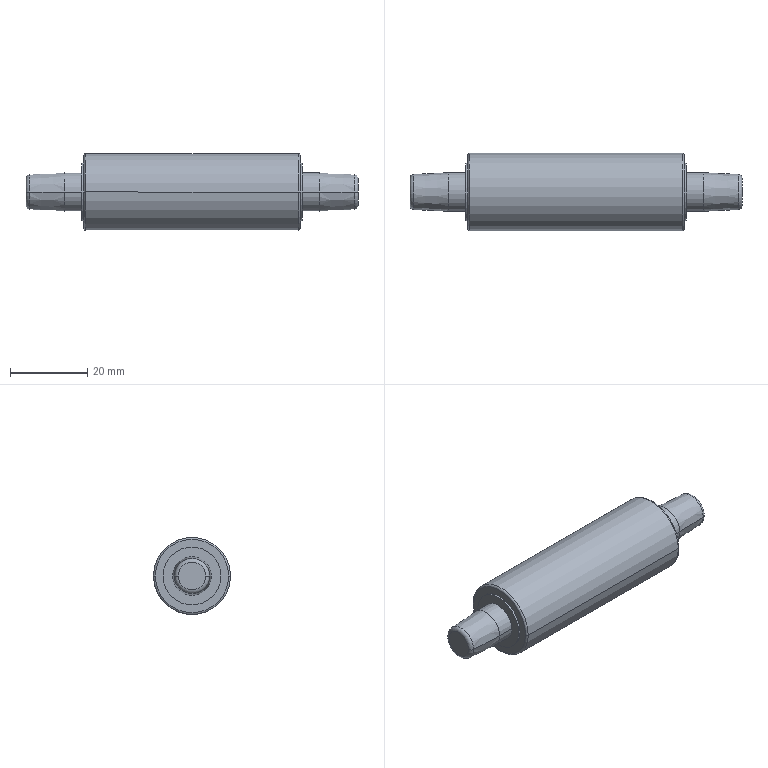Component | SolidWorks | RMS_20X400_03-1_RMS20X50_Piston-1 | 1 solid | 28 faces | box 86 x 20 x 20 mm | volume 19878 mm3 | cylinder 10 | torus 8 | plane 6 | cone 4 | commonest cylinder face diameters 10 x4 15 x4 20 x2
build123d program:
from build123d import *


with BuildPart() as part:
    # Sketch1 → Revolve1 (revolve)
    with BuildSketch(Plane.XY, mode=Mode.PRIVATE) as revolve1_sk:
        with BuildLine():
            Line((-15, 0), (-15, 3.549))
            ThreePointArc((-15, 3.549), (-14.725, 4.238), (-14.05, 4.548))
            Line((-14.05, 4.548), (-5, 5))
            Line((-5, 5), (-0.5, 5))
            Line((-0.5, 5), (-0.5, 7.5))
            Line((-0.5, 7.5), (0, 7.5))
            Line((0, 7.5), (0, 9.5))
            ThreePointArc((0, 9.5), (0.1464, 9.854), (0.5, 10))
            Line((0.5, 10), (55.5, 10))
            ThreePointArc((55.5, 10), (55.854, 9.854), (56, 9.5))
            Line((56, 9.5), (56, 7.5))
            Line((56, 7.5), (56.5, 7.5))
            Line((56.5, 7.5), (56.5, 5))
            Line((56.5, 5), (61, 5))
            Line((61, 5), (70.05, 4.548))
            ThreePointArc((70.05, 4.548), (70.725, 4.238), (71, 3.549))
            Line((71, 3.549), (71, 0))
            Line((71, 0), (-15, 0))
        make_face()
    revolve(revolve1_sk.sketch.rotate(Axis((71, 0, 0), (-1, 0, 0)), 270), axis=Axis((71, 0, 0), (-1, 0, 0)))


solid = part.part

# Placed as in the assembly
solid = solid.moved(Location((-0.1195, 21, 41.5), (0, 0, 0)))
STEP:
#1=CARTESIAN_POINT('',(2.791,0.9665,1.634));
#2=VERTEX_POINT('',#1);
#3=CARTESIAN_POINT('',(2.791,0.6871,1.634));
#4=VERTEX_POINT('',#3);
#5=CARTESIAN_POINT('',(2.791,0.8268,1.634));
#6=DIRECTION('',(-1.,0.,0.));
#7=DIRECTION('',(0.,1.,0.));
#8=AXIS2_PLACEMENT_3D('',#5,#6,#7);
#9=CIRCLE('',#8,0.1397);
#10=EDGE_CURVE('',#2,#4,#9,.T.);
#11=ORIENTED_EDGE('',*,*,#10,.T.);
#12=CARTESIAN_POINT('',(2.753,0.6477,1.634));
#13=VERTEX_POINT('',#12);
#14=CARTESIAN_POINT('',(2.751,0.6871,1.634));
#15=DIRECTION('',(-0.,0.,-1.));
#16=DIRECTION('',(0.,1.,0.));
#17=AXIS2_PLACEMENT_3D('',#14,#15,#16);
#18=CIRCLE('',#17,0.03937);
#19=EDGE_CURVE('',#4,#13,#18,.T.);
#20=ORIENTED_EDGE('',*,*,#19,.T.);
#21=CARTESIAN_POINT('',(2.753,1.006,1.634));
#22=VERTEX_POINT('',#21);
#23=CARTESIAN_POINT('',(2.753,0.8268,1.634));
#24=DIRECTION('',(-1.,0.,0.));
#25=DIRECTION('',(0.,1.,0.));
#26=AXIS2_PLACEMENT_3D('',#23,#24,#25);
#27=CIRCLE('',#26,0.179);
#28=EDGE_CURVE('',#22,#13,#27,.T.);
#29=ORIENTED_EDGE('',*,*,#28,.F.);
#30=CARTESIAN_POINT('',(2.751,0.9665,1.634));
#31=DIRECTION('',(0.,-0.,1.));
#32=DIRECTION('',(1.,0.,0.));
#33=AXIS2_PLACEMENT_3D('',#30,#31,#32);
#34=CIRCLE('',#33,0.03937);
#35=EDGE_CURVE('',#2,#22,#34,.T.);
#36=ORIENTED_EDGE('',*,*,#35,.F.);
#37=EDGE_LOOP('',(#11,#20,#29,#36));
#38=FACE_OUTER_BOUND('',#37,.T.);
#39=CARTESIAN_POINT('',(2.751,0.8268,1.634));
#40=DIRECTION('',(-1.,0.,0.));
#41=DIRECTION('',(0.,1.,-0.));
#42=AXIS2_PLACEMENT_3D('',#39,#40,#41);
#43=TOROIDAL_SURFACE('',#42,0.1397,0.03937);
#44=ADVANCED_FACE('',(#38),#43,.T.);
#45=ORIENTED_EDGE('',*,*,#28,.T.);
#46=CARTESIAN_POINT('',(2.397,0.6299,1.634));
#47=VERTEX_POINT('',#46);
#48=CARTESIAN_POINT('',(2.753,0.6477,1.634));
#49=DIRECTION('',(-0.9988,-0.04994,0.));
#50=VECTOR('',#49,39.37);
#51=LINE('',#48,#50);
#52=EDGE_CURVE('',#13,#47,#51,.T.);
#53=ORIENTED_EDGE('',*,*,#52,.T.);
#54=CARTESIAN_POINT('',(2.397,1.024,1.634));
#55=VERTEX_POINT('',#54);
#56=CARTESIAN_POINT('',(2.397,0.8268,1.634));
#57=DIRECTION('',(-1.,0.,0.));
#58=DIRECTION('',(0.,1.,0.));
#59=AXIS2_PLACEMENT_3D('',#56,#57,#58);
#60=CIRCLE('',#59,0.1969);
#61=EDGE_CURVE('',#55,#47,#60,.T.);
#62=ORIENTED_EDGE('',*,*,#61,.F.);
#63=CARTESIAN_POINT('',(2.753,1.006,1.634));
#64=DIRECTION('',(-0.9988,0.04994,0.));
#65=VECTOR('',#64,39.37);
#66=LINE('',#63,#65);
#67=EDGE_CURVE('',#22,#55,#66,.T.);
#68=ORIENTED_EDGE('',*,*,#67,.F.);
#69=EDGE_LOOP('',(#45,#53,#62,#68));
#70=FACE_OUTER_BOUND('',#69,.T.);
#71=CARTESIAN_POINT('',(2.753,0.8268,1.634));
#72=DIRECTION('',(-1.,0.,0.));
#73=DIRECTION('',(0.,1.,0.));
#74=AXIS2_PLACEMENT_3D('',#71,#72,#73);
#75=CONICAL_SURFACE('',#74,0.179,0.04996);
#76=ADVANCED_FACE('',(#70),#75,.T.);
#77=ORIENTED_EDGE('',*,*,#61,.T.);
#78=CARTESIAN_POINT('',(2.22,0.6299,1.634));
#79=VERTEX_POINT('',#78);
#80=CARTESIAN_POINT('',(2.791,0.6299,1.634));
#81=DIRECTION('',(-1.,0.,0.));
#82=VECTOR('',#81,39.37);
#83=LINE('',#80,#82);
#84=EDGE_CURVE('',#47,#79,#83,.T.);
#85=ORIENTED_EDGE('',*,*,#84,.T.);
#86=CARTESIAN_POINT('',(2.22,1.024,1.634));
#87=VERTEX_POINT('',#86);
#88=CARTESIAN_POINT('',(2.22,0.8268,1.634));
#89=DIRECTION('',(-1.,0.,0.));
#90=DIRECTION('',(0.,1.,0.));
#91=AXIS2_PLACEMENT_3D('',#88,#89,#90);
#92=CIRCLE('',#91,0.1969);
#93=EDGE_CURVE('',#87,#79,#92,.T.);
#94=ORIENTED_EDGE('',*,*,#93,.F.);
#95=CARTESIAN_POINT('',(2.791,1.024,1.634));
#96=DIRECTION('',(-1.,0.,0.));
#97=VECTOR('',#96,39.37);
#98=LINE('',#95,#97);
#99=EDGE_CURVE('',#55,#87,#98,.T.);
#100=ORIENTED_EDGE('',*,*,#99,.F.);
#101=EDGE_LOOP('',(#77,#85,#94,#100));
#102=FACE_OUTER_BOUND('',#101,.T.);
#103=CARTESIAN_POINT('',(2.791,0.8268,1.634));
#104=DIRECTION('',(-1.,0.,0.));
#105=DIRECTION('',(0.,1.,0.));
#106=AXIS2_PLACEMENT_3D('',#103,#104,#105);
#107=CYLINDRICAL_SURFACE('',#106,0.1969);
#108=ADVANCED_FACE('',(#102),#107,.T.);
#109=CARTESIAN_POINT('',(2.22,1.122,1.634));
#110=VERTEX_POINT('',#109);
#111=CARTESIAN_POINT('',(2.22,0.5315,1.634));
#112=VERTEX_POINT('',#111);
#113=CARTESIAN_POINT('',(2.22,0.8268,1.634));
#114=DIRECTION('',(-1.,0.,0.));
#115=DIRECTION('',(0.,1.,0.));
#116=AXIS2_PLACEMENT_3D('',#113,#114,#115);
#117=CIRCLE('',#116,0.2953);
#118=EDGE_CURVE('',#110,#112,#117,.T.);
#119=ORIENTED_EDGE('',*,*,#118,.T.);
#120=CARTESIAN_POINT('',(2.2,0.5315,1.634));
#121=VERTEX_POINT('',#120);
#122=CARTESIAN_POINT('',(2.791,0.5315,1.634));
#123=DIRECTION('',(-1.,0.,0.));
#124=VECTOR('',#123,39.37);
#125=LINE('',#122,#124);
#126=EDGE_CURVE('',#112,#121,#125,.T.);
#127=ORIENTED_EDGE('',*,*,#126,.T.);
#128=CARTESIAN_POINT('',(2.2,1.122,1.634));
#129=VERTEX_POINT('',#128);
#130=CARTESIAN_POINT('',(2.2,0.8268,1.634));
#131=DIRECTION('',(-1.,0.,0.));
#132=DIRECTION('',(0.,1.,0.));
#133=AXIS2_PLACEMENT_3D('',#130,#131,#132);
#134=CIRCLE('',#133,0.2953);
#135=EDGE_CURVE('',#129,#121,#134,.T.);
#136=ORIENTED_EDGE('',*,*,#135,.F.);
#137=CARTESIAN_POINT('',(2.791,1.122,1.634));
#138=DIRECTION('',(-1.,0.,0.));
#139=VECTOR('',#138,39.37);
#140=LINE('',#137,#139);
#141=EDGE_CURVE('',#110,#129,#140,.T.);
#142=ORIENTED_EDGE('',*,*,#141,.F.);
#143=EDGE_LOOP('',(#119,#127,#136,#142));
#144=FACE_OUTER_BOUND('',#143,.T.);
#145=CARTESIAN_POINT('',(2.791,0.8268,1.634));
#146=DIRECTION('',(-1.,0.,0.));
#147=DIRECTION('',(0.,1.,0.));
#148=AXIS2_PLACEMENT_3D('',#145,#146,#147);
#149=CYLINDRICAL_SURFACE('',#148,0.2953);
#150=ADVANCED_FACE('',(#144),#149,.T.);
#151=CARTESIAN_POINT('',(2.2,1.201,1.634));
#152=VERTEX_POINT('',#151);
#153=CARTESIAN_POINT('',(2.2,0.4528,1.634));
#154=VERTEX_POINT('',#153);
#155=CARTESIAN_POINT('',(2.2,0.8268,1.634));
#156=DIRECTION('',(-1.,0.,0.));
#157=DIRECTION('',(0.,1.,0.));
#158=AXIS2_PLACEMENT_3D('',#155,#156,#157);
#159=CIRCLE('',#158,0.374);
#160=EDGE_CURVE('',#152,#154,#159,.T.);
#161=ORIENTED_EDGE('',*,*,#160,.T.);
#162=CARTESIAN_POINT('',(2.18,0.4331,1.634));
#163=VERTEX_POINT('',#162);
#164=CARTESIAN_POINT('',(2.18,0.4528,1.634));
#165=DIRECTION('',(-0.,0.,-1.));
#166=DIRECTION('',(0.,1.,0.));
#167=AXIS2_PLACEMENT_3D('',#164,#165,#166);
#168=CIRCLE('',#167,0.01969);
#169=EDGE_CURVE('',#154,#163,#168,.T.);
#170=ORIENTED_EDGE('',*,*,#169,.T.);
#171=CARTESIAN_POINT('',(2.18,1.22,1.634));
#172=VERTEX_POINT('',#171);
#173=CARTESIAN_POINT('',(2.18,0.8268,1.634));
#174=DIRECTION('',(-1.,0.,0.));
#175=DIRECTION('',(0.,1.,0.));
#176=AXIS2_PLACEMENT_3D('',#173,#174,#175);
#177=CIRCLE('',#176,0.3937);
#178=EDGE_CURVE('',#172,#163,#177,.T.);
#179=ORIENTED_EDGE('',*,*,#178,.F.);
#180=CARTESIAN_POINT('',(2.18,1.201,1.634));
#181=DIRECTION('',(0.,-0.,1.));
#182=DIRECTION('',(1.,0.,0.));
#183=AXIS2_PLACEMENT_3D('',#180,#181,#182);
#184=CIRCLE('',#183,0.01969);
#185=EDGE_CURVE('',#152,#172,#184,.T.);
#186=ORIENTED_EDGE('',*,*,#185,.F.);
#187=EDGE_LOOP('',(#161,#170,#179,#186));
#188=FACE_OUTER_BOUND('',#187,.T.);
#189=CARTESIAN_POINT('',(2.18,0.8268,1.634));
#190=DIRECTION('',(-1.,0.,0.));
#191=DIRECTION('',(0.,1.,-0.));
#192=AXIS2_PLACEMENT_3D('',#189,#190,#191);
#193=TOROIDAL_SURFACE('',#192,0.374,0.01969);
#194=ADVANCED_FACE('',(#188),#193,.T.);
#195=ORIENTED_EDGE('',*,*,#178,.T.);
#196=CARTESIAN_POINT('',(0.01498,0.4331,1.634));
#197=VERTEX_POINT('',#196);
#198=CARTESIAN_POINT('',(2.791,0.4331,1.634));
#199=DIRECTION('',(-1.,0.,0.));
#200=VECTOR('',#199,39.37);
#201=LINE('',#198,#200);
#202=EDGE_CURVE('',#163,#197,#201,.T.);
#203=ORIENTED_EDGE('',*,*,#202,.T.);
#204=CARTESIAN_POINT('',(0.01498,1.22,1.634));
#205=VERTEX_POINT('',#204);
#206=CARTESIAN_POINT('',(0.01498,0.8268,1.634));
#207=DIRECTION('',(-1.,0.,0.));
#208=DIRECTION('',(0.,1.,0.));
#209=AXIS2_PLACEMENT_3D('',#206,#207,#208);
#210=CIRCLE('',#209,0.3937);
#211=EDGE_CURVE('',#205,#197,#210,.T.);
#212=ORIENTED_EDGE('',*,*,#211,.F.);
#213=CARTESIAN_POINT('',(2.791,1.22,1.634));
#214=DIRECTION('',(-1.,0.,0.));
#215=VECTOR('',#214,39.37);
#216=LINE('',#213,#215);
#217=EDGE_CURVE('',#172,#205,#216,.T.);
#218=ORIENTED_EDGE('',*,*,#217,.F.);
#219=EDGE_LOOP('',(#195,#203,#212,#218));
#220=FACE_OUTER_BOUND('',#219,.T.);
#221=CARTESIAN_POINT('',(2.791,0.8268,1.634));
#222=DIRECTION('',(-1.,0.,0.));
#223=DIRECTION('',(0.,1.,0.));
#224=AXIS2_PLACEMENT_3D('',#221,#222,#223);
#225=CYLINDRICAL_SURFACE('',#224,0.3937);
#226=ADVANCED_FACE('',(#220),#225,.T.);
#227=ORIENTED_EDGE('',*,*,#211,.T.);
#228=CARTESIAN_POINT('',(-0.004703,0.4528,1.634));
#229=VERTEX_POINT('',#228);
#230=CARTESIAN_POINT('',(0.01498,0.4528,1.634));
#231=DIRECTION('',(-0.,0.,-1.));
#232=DIRECTION('',(0.,1.,0.));
#233=AXIS2_PLACEMENT_3D('',#230,#231,#232);
#234=CIRCLE('',#233,0.01969);
#235=EDGE_CURVE('',#197,#229,#234,.T.);
#236=ORIENTED_EDGE('',*,*,#235,.T.);
#237=CARTESIAN_POINT('',(-0.004703,1.201,1.634));
#238=VERTEX_POINT('',#237);
#239=CARTESIAN_POINT('',(-0.004703,0.8268,1.634));
#240=DIRECTION('',(-1.,0.,0.));
#241=DIRECTION('',(0.,1.,0.));
#242=AXIS2_PLACEMENT_3D('',#239,#240,#241);
#243=CIRCLE('',#242,0.374);
#244=EDGE_CURVE('',#238,#229,#243,.T.);
#245=ORIENTED_EDGE('',*,*,#244,.F.);
#246=CARTESIAN_POINT('',(0.01498,1.201,1.634));
#247=DIRECTION('',(0.,-0.,1.));
#248=DIRECTION('',(1.,0.,0.));
#249=AXIS2_PLACEMENT_3D('',#246,#247,#248);
#250=CIRCLE('',#249,0.01969);
#251=EDGE_CURVE('',#205,#238,#250,.T.);
#252=ORIENTED_EDGE('',*,*,#251,.F.);
#253=EDGE_LOOP('',(#227,#236,#245,#252));
#254=FACE_OUTER_BOUND('',#253,.T.);
#255=CARTESIAN_POINT('',(0.01498,0.8268,1.634));
#256=DIRECTION('',(-1.,0.,0.));
#257=DIRECTION('',(0.,1.,-0.));
#258=AXIS2_PLACEMENT_3D('',#255,#256,#257);
#259=TOROIDAL_SURFACE('',#258,0.374,0.01969);
#260=ADVANCED_FACE('',(#254),#259,.T.);
#261=CARTESIAN_POINT('',(-0.004703,1.122,1.634));
#262=VERTEX_POINT('',#261);
#263=CARTESIAN_POINT('',(-0.004703,0.5315,1.634));
#264=VERTEX_POINT('',#263);
#265=CARTESIAN_POINT('',(-0.004703,0.8268,1.634));
#266=DIRECTION('',(-1.,0.,0.));
#267=DIRECTION('',(0.,1.,0.));
#268=AXIS2_PLACEMENT_3D('',#265,#266,#267);
#269=CIRCLE('',#268,0.2953);
#270=EDGE_CURVE('',#262,#264,#269,.T.);
#271=ORIENTED_EDGE('',*,*,#270,.T.);
#272=CARTESIAN_POINT('',(-0.02439,0.5315,1.634));
#273=VERTEX_POINT('',#272);
#274=CARTESIAN_POINT('',(2.791,0.5315,1.634));
#275=DIRECTION('',(-1.,0.,0.));
#276=VECTOR('',#275,39.37);
#277=LINE('',#274,#276);
#278=EDGE_CURVE('',#264,#273,#277,.T.);
#279=ORIENTED_EDGE('',*,*,#278,.T.);
#280=CARTESIAN_POINT('',(-0.02439,1.122,1.634));
#281=VERTEX_POINT('',#280);
#282=CARTESIAN_POINT('',(-0.02439,0.8268,1.634));
#283=DIRECTION('',(-1.,0.,0.));
#284=DIRECTION('',(0.,1.,0.));
#285=AXIS2_PLACEMENT_3D('',#282,#283,#284);
#286=CIRCLE('',#285,0.2953);
#287=EDGE_CURVE('',#281,#273,#286,.T.);
#288=ORIENTED_EDGE('',*,*,#287,.F.);
#289=CARTESIAN_POINT('',(2.791,1.122,1.634));
#290=DIRECTION('',(-1.,0.,0.));
#291=VECTOR('',#290,39.37);
#292=LINE('',#289,#291);
#293=EDGE_CURVE('',#262,#281,#292,.T.);
#294=ORIENTED_EDGE('',*,*,#293,.F.);
#295=EDGE_LOOP('',(#271,#279,#288,#294));
#296=FACE_OUTER_BOUND('',#295,.T.);
#297=CARTESIAN_POINT('',(2.791,0.8268,1.634));
#298=DIRECTION('',(-1.,0.,0.));
#299=DIRECTION('',(0.,1.,0.));
#300=AXIS2_PLACEMENT_3D('',#297,#298,#299);
#301=CYLINDRICAL_SURFACE('',#300,0.2953);
#302=ADVANCED_FACE('',(#296),#301,.T.);
#303=CARTESIAN_POINT('',(-0.02439,1.024,1.634));
#304=VERTEX_POINT('',#303);
#305=CARTESIAN_POINT('',(-0.02439,0.6299,1.634));
#306=VERTEX_POINT('',#305);
#307=CARTESIAN_POINT('',(-0.02439,0.8268,1.634));
#308=DIRECTION('',(-1.,0.,0.));
#309=DIRECTION('',(0.,1.,0.));
#310=AXIS2_PLACEMENT_3D('',#307,#308,#309);
#311=CIRCLE('',#310,0.1969);
#312=EDGE_CURVE('',#304,#306,#311,.T.);
#313=ORIENTED_EDGE('',*,*,#312,.T.);
#314=CARTESIAN_POINT('',(-0.2016,0.6299,1.634));
#315=VERTEX_POINT('',#314);
#316=CARTESIAN_POINT('',(2.791,0.6299,1.634));
#317=DIRECTION('',(-1.,0.,0.));
#318=VECTOR('',#317,39.37);
#319=LINE('',#316,#318);
#320=EDGE_CURVE('',#306,#315,#319,.T.);
#321=ORIENTED_EDGE('',*,*,#320,.T.);
#322=CARTESIAN_POINT('',(-0.2016,1.024,1.634));
#323=VERTEX_POINT('',#322);
#324=CARTESIAN_POINT('',(-0.2016,0.8268,1.634));
#325=DIRECTION('',(-1.,0.,0.));
#326=DIRECTION('',(0.,1.,0.));
#327=AXIS2_PLACEMENT_3D('',#324,#325,#326);
#328=CIRCLE('',#327,0.1969);
#329=EDGE_CURVE('',#323,#315,#328,.T.);
#330=ORIENTED_EDGE('',*,*,#329,.F.);
#331=CARTESIAN_POINT('',(2.791,1.024,1.634));
#332=DIRECTION('',(-1.,0.,0.));
#333=VECTOR('',#332,39.37);
#334=LINE('',#331,#333);
#335=EDGE_CURVE('',#304,#323,#334,.T.);
#336=ORIENTED_EDGE('',*,*,#335,.F.);
#337=EDGE_LOOP('',(#313,#321,#330,#336));
#338=FACE_OUTER_BOUND('',#337,.T.);
#339=CARTESIAN_POINT('',(2.791,0.8268,1.634));
#340=DIRECTION('',(-1.,0.,0.));
#341=DIRECTION('',(0.,1.,0.));
#342=AXIS2_PLACEMENT_3D('',#339,#340,#341);
#343=CYLINDRICAL_SURFACE('',#342,0.1969);
#344=ADVANCED_FACE('',(#338),#343,.T.);
#345=CARTESIAN_POINT('',(-0.5579,1.006,1.634));
#346=VERTEX_POINT('',#345);
#347=CARTESIAN_POINT('',(-0.5579,0.6477,1.634));
#348=VERTEX_POINT('',#347);
#349=CARTESIAN_POINT('',(-0.5579,0.8268,1.634));
#350=DIRECTION('',(-1.,0.,0.));
#351=DIRECTION('',(0.,1.,0.));
#352=AXIS2_PLACEMENT_3D('',#349,#350,#351);
#353=CIRCLE('',#352,0.179);
#354=EDGE_CURVE('',#346,#348,#353,.T.);
#355=ORIENTED_EDGE('',*,*,#354,.F.);
#356=CARTESIAN_POINT('',(-0.2016,1.024,1.634));
#357=DIRECTION('',(0.9988,0.04994,-0.));
#358=VECTOR('',#357,39.37);
#359=LINE('',#356,#358);
#360=EDGE_CURVE('',#346,#323,#359,.T.);
#361=ORIENTED_EDGE('',*,*,#360,.T.);
#362=ORIENTED_EDGE('',*,*,#329,.T.);
#363=CARTESIAN_POINT('',(-0.2016,0.6299,1.634));
#364=DIRECTION('',(0.9988,-0.04994,-0.));
#365=VECTOR('',#364,39.37);
#366=LINE('',#363,#365);
#367=EDGE_CURVE('',#348,#315,#366,.T.);
#368=ORIENTED_EDGE('',*,*,#367,.F.);
#369=EDGE_LOOP('',(#355,#361,#362,#368));
#370=FACE_OUTER_BOUND('',#369,.T.);
#371=CARTESIAN_POINT('',(-0.2016,0.8268,1.634));
#372=DIRECTION('',(1.,-0.,-0.));
#373=DIRECTION('',(-0.,-1.,0.));
#374=AXIS2_PLACEMENT_3D('',#371,#372,#373);
#375=CONICAL_SURFACE('',#374,0.1969,0.04996);
#376=ADVANCED_FACE('',(#370),#375,.T.);
#377=ORIENTED_EDGE('',*,*,#354,.T.);
#378=CARTESIAN_POINT('',(-0.5953,0.6871,1.634));
#379=VERTEX_POINT('',#378);
#380=CARTESIAN_POINT('',(-0.5559,0.6871,1.634));
#381=DIRECTION('',(-0.,0.,-1.));
#382=DIRECTION('',(0.,1.,0.));
#383=AXIS2_PLACEMENT_3D('',#380,#381,#382);
#384=CIRCLE('',#383,0.03937);
#385=EDGE_CURVE('',#348,#379,#384,.T.);
#386=ORIENTED_EDGE('',*,*,#385,.T.);
#387=CARTESIAN_POINT('',(-0.5953,0.9665,1.634));
#388=VERTEX_POINT('',#387);
#389=CARTESIAN_POINT('',(-0.5953,0.8268,1.634));
#390=DIRECTION('',(-1.,0.,0.));
#391=DIRECTION('',(0.,1.,0.));
#392=AXIS2_PLACEMENT_3D('',#389,#390,#391);
#393=CIRCLE('',#392,0.1397);
#394=EDGE_CURVE('',#388,#379,#393,.T.);
#395=ORIENTED_EDGE('',*,*,#394,.F.);
#396=CARTESIAN_POINT('',(-0.5559,0.9665,1.634));
#397=DIRECTION('',(0.,-0.,1.));
#398=DIRECTION('',(1.,0.,0.));
#399=AXIS2_PLACEMENT_3D('',#396,#397,#398);
#400=CIRCLE('',#399,0.03937);
#401=EDGE_CURVE('',#346,#388,#400,.T.);
#402=ORIENTED_EDGE('',*,*,#401,.F.);
#403=EDGE_LOOP('',(#377,#386,#395,#402));
#404=FACE_OUTER_BOUND('',#403,.T.);
#405=CARTESIAN_POINT('',(-0.5559,0.8268,1.634));
#406=DIRECTION('',(-1.,0.,0.));
#407=DIRECTION('',(0.,1.,-0.));
#408=AXIS2_PLACEMENT_3D('',#405,#406,#407);
#409=TOROIDAL_SURFACE('',#408,0.1397,0.03937);
#410=ADVANCED_FACE('',(#404),#409,.T.);
#411=ORIENTED_EDGE('',*,*,#394,.T.);
#412=CARTESIAN_POINT('',(-0.5953,0.8268,1.634));
#413=DIRECTION('',(-1.,0.,0.));
#414=DIRECTION('',(0.,1.,0.));
#415=AXIS2_PLACEMENT_3D('',#412,#413,#414);
#416=CIRCLE('',#415,0.1397);
#417=EDGE_CURVE('',#379,#388,#416,.T.);
#418=ORIENTED_EDGE('',*,*,#417,.T.);
#419=EDGE_LOOP('',(#411,#418));
#420=FACE_OUTER_BOUND('',#419,.T.);
#421=CARTESIAN_POINT('',(-0.5953,0.8268,1.634));
#422=DIRECTION('',(1.,-0.,-0.));
#423=DIRECTION('',(-0.,-1.,-0.));
#424=AXIS2_PLACEMENT_3D('',#421,#422,#423);
#425=PLANE('',#424);
#426=ADVANCED_FACE('',(#420),#425,.F.);
#427=ORIENTED_EDGE('',*,*,#385,.F.);
#428=CARTESIAN_POINT('',(-0.5579,0.8268,1.634));
#429=DIRECTION('',(-1.,0.,0.));
#430=DIRECTION('',(0.,1.,0.));
#431=AXIS2_PLACEMENT_3D('',#428,#429,#430);
#432=CIRCLE('',#431,0.179);
#433=EDGE_CURVE('',#348,#346,#432,.T.);
#434=ORIENTED_EDGE('',*,*,#433,.T.);
#435=ORIENTED_EDGE('',*,*,#401,.T.);
#436=ORIENTED_EDGE('',*,*,#417,.F.);
#437=EDGE_LOOP('',(#427,#434,#435,#436));
#438=FACE_OUTER_BOUND('',#437,.T.);
#439=CARTESIAN_POINT('',(-0.5559,0.8268,1.634));
#440=DIRECTION('',(-1.,0.,0.));
#441=DIRECTION('',(0.,1.,-0.));
#442=AXIS2_PLACEMENT_3D('',#439,#440,#441);
#443=TOROIDAL_SURFACE('',#442,0.1397,0.03937);
#444=ADVANCED_FACE('',(#438),#443,.T.);
#445=ORIENTED_EDGE('',*,*,#360,.F.);
#446=ORIENTED_EDGE('',*,*,#433,.F.);
#447=ORIENTED_EDGE('',*,*,#367,.T.);
#448=CARTESIAN_POINT('',(-0.2016,0.8268,1.634));
#449=DIRECTION('',(-1.,0.,0.));
#450=DIRECTION('',(0.,1.,0.));
#451=AXIS2_PLACEMENT_3D('',#448,#449,#450);
#452=CIRCLE('',#451,0.1969);
#453=EDGE_CURVE('',#315,#323,#452,.T.);
#454=ORIENTED_EDGE('',*,*,#453,.T.);
#455=EDGE_LOOP('',(#445,#446,#447,#454));
#456=FACE_OUTER_BOUND('',#455,.T.);
#457=CARTESIAN_POINT('',(-0.2016,0.8268,1.634));
#458=DIRECTION('',(1.,-0.,-0.));
#459=DIRECTION('',(-0.,-1.,0.));
#460=AXIS2_PLACEMENT_3D('',#457,#458,#459);
#461=CONICAL_SURFACE('',#460,0.1969,0.04996);
#462=ADVANCED_FACE('',(#456),#461,.T.);
#463=ORIENTED_EDGE('',*,*,#320,.F.);
#464=CARTESIAN_POINT('',(-0.02439,0.8268,1.634));
#465=DIRECTION('',(-1.,0.,0.));
#466=DIRECTION('',(0.,1.,0.));
#467=AXIS2_PLACEMENT_3D('',#464,#465,#466);
#468=CIRCLE('',#467,0.1969);
#469=EDGE_CURVE('',#306,#304,#468,.T.);
#470=ORIENTED_EDGE('',*,*,#469,.T.);
#471=ORIENTED_EDGE('',*,*,#335,.T.);
#472=ORIENTED_EDGE('',*,*,#453,.F.);
#473=EDGE_LOOP('',(#463,#470,#471,#472));
#474=FACE_OUTER_BOUND('',#473,.T.);
#475=CARTESIAN_POINT('',(2.791,0.8268,1.634));
#476=DIRECTION('',(-1.,0.,0.));
#477=DIRECTION('',(0.,1.,0.));
#478=AXIS2_PLACEMENT_3D('',#475,#476,#477);
#479=CYLINDRICAL_SURFACE('',#478,0.1969);
#480=ADVANCED_FACE('',(#474),#479,.T.);
#481=ORIENTED_EDGE('',*,*,#312,.F.);
#482=ORIENTED_EDGE('',*,*,#469,.F.);
#483=EDGE_LOOP('',(#481,#482));
#484=FACE_BOUND('',#483,.T.);
#485=ORIENTED_EDGE('',*,*,#287,.T.);
#486=CARTESIAN_POINT('',(-0.02439,0.8268,1.634));
#487=DIRECTION('',(-1.,0.,0.));
#488=DIRECTION('',(0.,1.,0.));
#489=AXIS2_PLACEMENT_3D('',#486,#487,#488);
#490=CIRCLE('',#489,0.2953);
#491=EDGE_CURVE('',#273,#281,#490,.T.);
#492=ORIENTED_EDGE('',*,*,#491,.T.);
#493=EDGE_LOOP('',(#485,#492));
#494=FACE_OUTER_BOUND('',#493,.T.);
#495=CARTESIAN_POINT('',(-0.02439,0.8268,1.437));
#496=DIRECTION('',(1.,-0.,-0.));
#497=DIRECTION('',(-0.,-1.,-0.));
#498=AXIS2_PLACEMENT_3D('',#495,#496,#497);
#499=PLANE('',#498);
#500=ADVANCED_FACE('',(#484,#494),#499,.F.);
#501=ORIENTED_EDGE('',*,*,#278,.F.);
#502=CARTESIAN_POINT('',(-0.004703,0.8268,1.634));
#503=DIRECTION('',(-1.,0.,0.));
#504=DIRECTION('',(0.,1.,0.));
#505=AXIS2_PLACEMENT_3D('',#502,#503,#504);
#506=CIRCLE('',#505,0.2953);
#507=EDGE_CURVE('',#264,#262,#506,.T.);
#508=ORIENTED_EDGE('',*,*,#507,.T.);
#509=ORIENTED_EDGE('',*,*,#293,.T.);
#510=ORIENTED_EDGE('',*,*,#491,.F.);
#511=EDGE_LOOP('',(#501,#508,#509,#510));
#512=FACE_OUTER_BOUND('',#511,.T.);
#513=CARTESIAN_POINT('',(2.791,0.8268,1.634));
#514=DIRECTION('',(-1.,0.,0.));
#515=DIRECTION('',(0.,1.,0.));
#516=AXIS2_PLACEMENT_3D('',#513,#514,#515);
#517=CYLINDRICAL_SURFACE('',#516,0.2953);
#518=ADVANCED_FACE('',(#512),#517,.T.);
#519=ORIENTED_EDGE('',*,*,#270,.F.);
#520=ORIENTED_EDGE('',*,*,#507,.F.);
#521=EDGE_LOOP('',(#519,#520));
#522=FACE_BOUND('',#521,.T.);
#523=ORIENTED_EDGE('',*,*,#244,.T.);
#524=CARTESIAN_POINT('',(-0.004703,0.8268,1.634));
#525=DIRECTION('',(-1.,0.,0.));
#526=DIRECTION('',(0.,1.,0.));
#527=AXIS2_PLACEMENT_3D('',#524,#525,#526);
#528=CIRCLE('',#527,0.374);
#529=EDGE_CURVE('',#229,#238,#528,.T.);
#530=ORIENTED_EDGE('',*,*,#529,.T.);
#531=EDGE_LOOP('',(#523,#530));
#532=FACE_OUTER_BOUND('',#531,.T.);
#533=CARTESIAN_POINT('',(-0.004703,0.8268,1.339));
#534=DIRECTION('',(1.,-0.,-0.));
#535=DIRECTION('',(-0.,-1.,-0.));
#536=AXIS2_PLACEMENT_3D('',#533,#534,#535);
#537=PLANE('',#536);
#538=ADVANCED_FACE('',(#522,#532),#537,.F.);
#539=ORIENTED_EDGE('',*,*,#235,.F.);
#540=CARTESIAN_POINT('',(0.01498,0.8268,1.634));
#541=DIRECTION('',(-1.,0.,0.));
#542=DIRECTION('',(0.,1.,0.));
#543=AXIS2_PLACEMENT_3D('',#540,#541,#542);
#544=CIRCLE('',#543,0.3937);
#545=EDGE_CURVE('',#197,#205,#544,.T.);
#546=ORIENTED_EDGE('',*,*,#545,.T.);
#547=ORIENTED_EDGE('',*,*,#251,.T.);
#548=ORIENTED_EDGE('',*,*,#529,.F.);
#549=EDGE_LOOP('',(#539,#546,#547,#548));
#550=FACE_OUTER_BOUND('',#549,.T.);
#551=CARTESIAN_POINT('',(0.01498,0.8268,1.634));
#552=DIRECTION('',(-1.,0.,0.));
#553=DIRECTION('',(0.,1.,-0.));
#554=AXIS2_PLACEMENT_3D('',#551,#552,#553);
#555=TOROIDAL_SURFACE('',#554,0.374,0.01969);
#556=ADVANCED_FACE('',(#550),#555,.T.);
#557=ORIENTED_EDGE('',*,*,#202,.F.);
#558=CARTESIAN_POINT('',(2.18,0.8268,1.634));
#559=DIRECTION('',(-1.,0.,0.));
#560=DIRECTION('',(0.,1.,0.));
#561=AXIS2_PLACEMENT_3D('',#558,#559,#560);
#562=CIRCLE('',#561,0.3937);
#563=EDGE_CURVE('',#163,#172,#562,.T.);
#564=ORIENTED_EDGE('',*,*,#563,.T.);
#565=ORIENTED_EDGE('',*,*,#217,.T.);
#566=ORIENTED_EDGE('',*,*,#545,.F.);
#567=EDGE_LOOP('',(#557,#564,#565,#566));
#568=FACE_OUTER_BOUND('',#567,.T.);
#569=CARTESIAN_POINT('',(2.791,0.8268,1.634));
#570=DIRECTION('',(-1.,0.,0.));
#571=DIRECTION('',(0.,1.,0.));
#572=AXIS2_PLACEMENT_3D('',#569,#570,#571);
#573=CYLINDRICAL_SURFACE('',#572,0.3937);
#574=ADVANCED_FACE('',(#568),#573,.T.);
#575=ORIENTED_EDGE('',*,*,#169,.F.);
#576=CARTESIAN_POINT('',(2.2,0.8268,1.634));
#577=DIRECTION('',(-1.,0.,0.));
#578=DIRECTION('',(0.,1.,0.));
#579=AXIS2_PLACEMENT_3D('',#576,#577,#578);
#580=CIRCLE('',#579,0.374);
#581=EDGE_CURVE('',#154,#152,#580,.T.);
#582=ORIENTED_EDGE('',*,*,#581,.T.);
#583=ORIENTED_EDGE('',*,*,#185,.T.);
#584=ORIENTED_EDGE('',*,*,#563,.F.);
#585=EDGE_LOOP('',(#575,#582,#583,#584));
#586=FACE_OUTER_BOUND('',#585,.T.);
#587=CARTESIAN_POINT('',(2.18,0.8268,1.634));
#588=DIRECTION('',(-1.,0.,0.));
#589=DIRECTION('',(0.,1.,-0.));
#590=AXIS2_PLACEMENT_3D('',#587,#588,#589);
#591=TOROIDAL_SURFACE('',#590,0.374,0.01969);
#592=ADVANCED_FACE('',(#586),#591,.T.);
#593=ORIENTED_EDGE('',*,*,#160,.F.);
#594=ORIENTED_EDGE('',*,*,#581,.F.);
#595=EDGE_LOOP('',(#593,#594));
#596=FACE_OUTER_BOUND('',#595,.T.);
#597=ORIENTED_EDGE('',*,*,#135,.T.);
#598=CARTESIAN_POINT('',(2.2,0.8268,1.634));
#599=DIRECTION('',(-1.,0.,0.));
#600=DIRECTION('',(0.,1.,0.));
#601=AXIS2_PLACEMENT_3D('',#598,#599,#600);
#602=CIRCLE('',#601,0.2953);
#603=EDGE_CURVE('',#121,#129,#602,.T.);
#604=ORIENTED_EDGE('',*,*,#603,.T.);
#605=EDGE_LOOP('',(#597,#604));
#606=FACE_BOUND('',#605,.T.);
#607=CARTESIAN_POINT('',(2.2,0.8268,1.26));
#608=DIRECTION('',(-1.,0.,0.));
#609=DIRECTION('',(0.,1.,0.));
#610=AXIS2_PLACEMENT_3D('',#607,#608,#609);
#611=PLANE('',#610);
#612=ADVANCED_FACE('',(#596,#606),#611,.F.);
#613=ORIENTED_EDGE('',*,*,#126,.F.);
#614=CARTESIAN_POINT('',(2.22,0.8268,1.634));
#615=DIRECTION('',(-1.,0.,0.));
#616=DIRECTION('',(0.,1.,0.));
#617=AXIS2_PLACEMENT_3D('',#614,#615,#616);
#618=CIRCLE('',#617,0.2953);
#619=EDGE_CURVE('',#112,#110,#618,.T.);
#620=ORIENTED_EDGE('',*,*,#619,.T.);
#621=ORIENTED_EDGE('',*,*,#141,.T.);
#622=ORIENTED_EDGE('',*,*,#603,.F.);
#623=EDGE_LOOP('',(#613,#620,#621,#622));
#624=FACE_OUTER_BOUND('',#623,.T.);
#625=CARTESIAN_POINT('',(2.791,0.8268,1.634));
#626=DIRECTION('',(-1.,0.,0.));
#627=DIRECTION('',(0.,1.,0.));
#628=AXIS2_PLACEMENT_3D('',#625,#626,#627);
#629=CYLINDRICAL_SURFACE('',#628,0.2953);
#630=ADVANCED_FACE('',(#624),#629,.T.);
#631=ORIENTED_EDGE('',*,*,#118,.F.);
#632=ORIENTED_EDGE('',*,*,#619,.F.);
#633=EDGE_LOOP('',(#631,#632));
#634=FACE_OUTER_BOUND('',#633,.T.);
#635=ORIENTED_EDGE('',*,*,#93,.T.);
#636=CARTESIAN_POINT('',(2.22,0.8268,1.634));
#637=DIRECTION('',(-1.,0.,0.));
#638=DIRECTION('',(0.,1.,0.));
#639=AXIS2_PLACEMENT_3D('',#636,#637,#638);
#640=CIRCLE('',#639,0.1969);
#641=EDGE_CURVE('',#79,#87,#640,.T.);
#642=ORIENTED_EDGE('',*,*,#641,.T.);
#643=EDGE_LOOP('',(#635,#642));
#644=FACE_BOUND('',#643,.T.);
#645=CARTESIAN_POINT('',(2.22,0.8268,1.339));
#646=DIRECTION('',(-1.,0.,0.));
#647=DIRECTION('',(0.,1.,0.));
#648=AXIS2_PLACEMENT_3D('',#645,#646,#647);
#649=PLANE('',#648);
#650=ADVANCED_FACE('',(#634,#644),#649,.F.);
#651=ORIENTED_EDGE('',*,*,#84,.F.);
#652=CARTESIAN_POINT('',(2.397,0.8268,1.634));
#653=DIRECTION('',(-1.,0.,0.));
#654=DIRECTION('',(0.,1.,0.));
#655=AXIS2_PLACEMENT_3D('',#652,#653,#654);
#656=CIRCLE('',#655,0.1969);
#657=EDGE_CURVE('',#47,#55,#656,.T.);
#658=ORIENTED_EDGE('',*,*,#657,.T.);
#659=ORIENTED_EDGE('',*,*,#99,.T.);
#660=ORIENTED_EDGE('',*,*,#641,.F.);
#661=EDGE_LOOP('',(#651,#658,#659,#660));
#662=FACE_OUTER_BOUND('',#661,.T.);
#663=CARTESIAN_POINT('',(2.791,0.8268,1.634));
#664=DIRECTION('',(-1.,0.,0.));
#665=DIRECTION('',(0.,1.,0.));
#666=AXIS2_PLACEMENT_3D('',#663,#664,#665);
#667=CYLINDRICAL_SURFACE('',#666,0.1969);
#668=ADVANCED_FACE('',(#662),#667,.T.);
#669=ORIENTED_EDGE('',*,*,#52,.F.);
#670=CARTESIAN_POINT('',(2.753,0.8268,1.634));
#671=DIRECTION('',(-1.,0.,0.));
#672=DIRECTION('',(0.,1.,0.));
#673=AXIS2_PLACEMENT_3D('',#670,#671,#672);
#674=CIRCLE('',#673,0.179);
#675=EDGE_CURVE('',#13,#22,#674,.T.);
#676=ORIENTED_EDGE('',*,*,#675,.T.);
#677=ORIENTED_EDGE('',*,*,#67,.T.);
#678=ORIENTED_EDGE('',*,*,#657,.F.);
#679=EDGE_LOOP('',(#669,#676,#677,#678));
#680=FACE_OUTER_BOUND('',#679,.T.);
#681=CARTESIAN_POINT('',(2.753,0.8268,1.634));
#682=DIRECTION('',(-1.,0.,0.));
#683=DIRECTION('',(0.,1.,0.));
#684=AXIS2_PLACEMENT_3D('',#681,#682,#683);
#685=CONICAL_SURFACE('',#684,0.179,0.04996);
#686=ADVANCED_FACE('',(#680),#685,.T.);
#687=ORIENTED_EDGE('',*,*,#19,.F.);
#688=CARTESIAN_POINT('',(2.791,0.8268,1.634));
#689=DIRECTION('',(-1.,0.,0.));
#690=DIRECTION('',(0.,1.,0.));
#691=AXIS2_PLACEMENT_3D('',#688,#689,#690);
#692=CIRCLE('',#691,0.1397);
#693=EDGE_CURVE('',#4,#2,#692,.T.);
#694=ORIENTED_EDGE('',*,*,#693,.T.);
#695=ORIENTED_EDGE('',*,*,#35,.T.);
#696=ORIENTED_EDGE('',*,*,#675,.F.);
#697=EDGE_LOOP('',(#687,#694,#695,#696));
#698=FACE_OUTER_BOUND('',#697,.T.);
#699=CARTESIAN_POINT('',(2.751,0.8268,1.634));
#700=DIRECTION('',(-1.,0.,0.));
#701=DIRECTION('',(0.,1.,-0.));
#702=AXIS2_PLACEMENT_3D('',#699,#700,#701);
#703=TOROIDAL_SURFACE('',#702,0.1397,0.03937);
#704=ADVANCED_FACE('',(#698),#703,.T.);
#705=ORIENTED_EDGE('',*,*,#10,.F.);
#706=ORIENTED_EDGE('',*,*,#693,.F.);
#707=EDGE_LOOP('',(#705,#706));
#708=FACE_OUTER_BOUND('',#707,.T.);
#709=CARTESIAN_POINT('',(2.791,0.8268,1.494));
#710=DIRECTION('',(-1.,0.,0.));
#711=DIRECTION('',(0.,1.,0.));
#712=AXIS2_PLACEMENT_3D('',#709,#710,#711);
#713=PLANE('',#712);
#714=ADVANCED_FACE('',(#708),#713,.F.);
#715=CLOSED_SHELL('',(#44,#76,#108,#150,#194,#226,#260,#302,#344,#376,#410,#426,#444,#462,#480,#500,#518,#538,#556,#574,#592,#612,#630,#650,#668,#686,#704,#714));
#716=MANIFOLD_SOLID_BREP('',#715);
#717=CARTESIAN_POINT('',(0.,0.,0.));
#718=DIRECTION('',(0.,0.,1.));
#719=DIRECTION('',(1.,0.,0.));
#720=AXIS2_PLACEMENT_3D('',#717,#718,#719);
#721=(LENGTH_UNIT()NAMED_UNIT(*)SI_UNIT($,.METRE.));
#722=LENGTH_MEASURE_WITH_UNIT(LENGTH_MEASURE(0.0254),#721);
#723=DIMENSIONAL_EXPONENTS(1.,0.,0.,0.,0.,0.,0.);
#724=(CONVERSION_BASED_UNIT('',#722)LENGTH_UNIT()NAMED_UNIT(#723));
#725=UNCERTAINTY_MEASURE_WITH_UNIT(LENGTH_MEASURE(0.00001),#724,'','');
#726=(NAMED_UNIT(*)PLANE_ANGLE_UNIT()SI_UNIT($,.RADIAN.));
#727=(NAMED_UNIT(*)SI_UNIT($,.STERADIAN.)SOLID_ANGLE_UNIT());
#728=(GEOMETRIC_REPRESENTATION_CONTEXT(3)GLOBAL_UNCERTAINTY_ASSIGNED_CONTEXT((#725))GLOBAL_UNIT_ASSIGNED_CONTEXT((#724,#726,#727))REPRESENTATION_CONTEXT('',''));
#729=ADVANCED_BREP_SHAPE_REPRESENTATION('',(#716,#720),#728);
#730=COLOUR_RGB('',0.7922,0.8196,0.9333);
#731=FILL_AREA_STYLE_COLOUR('',#730);
#732=FILL_AREA_STYLE('',(#731));
#733=SURFACE_STYLE_FILL_AREA(#732);
#734=SURFACE_SIDE_STYLE('',(#733));
#735=SURFACE_STYLE_USAGE(.BOTH.,#734);
#736=PRESENTATION_STYLE_ASSIGNMENT((#735));
#737=STYLED_ITEM('',(#736),#716);
#738=(LENGTH_UNIT()NAMED_UNIT(*)SI_UNIT($,.METRE.));
#739=LENGTH_MEASURE_WITH_UNIT(LENGTH_MEASURE(0.0254),#738);
#740=DIMENSIONAL_EXPONENTS(1.,0.,0.,0.,0.,0.,0.);
#741=(CONVERSION_BASED_UNIT('',#739)LENGTH_UNIT()NAMED_UNIT(#740));
#742=UNCERTAINTY_MEASURE_WITH_UNIT(LENGTH_MEASURE(0.00001),#741,'','');
#743=(NAMED_UNIT(*)PLANE_ANGLE_UNIT()SI_UNIT($,.RADIAN.));
#744=(NAMED_UNIT(*)SI_UNIT($,.STERADIAN.)SOLID_ANGLE_UNIT());
#745=(GEOMETRIC_REPRESENTATION_CONTEXT(3)GLOBAL_UNCERTAINTY_ASSIGNED_CONTEXT((#742))GLOBAL_UNIT_ASSIGNED_CONTEXT((#741,#743,#744))REPRESENTATION_CONTEXT('',''));
#746=MECHANICAL_DESIGN_GEOMETRIC_PRESENTATION_REPRESENTATION('',(#737),#745);
#747=PRESENTATION_LAYER_ASSIGNMENT('','',(#737));